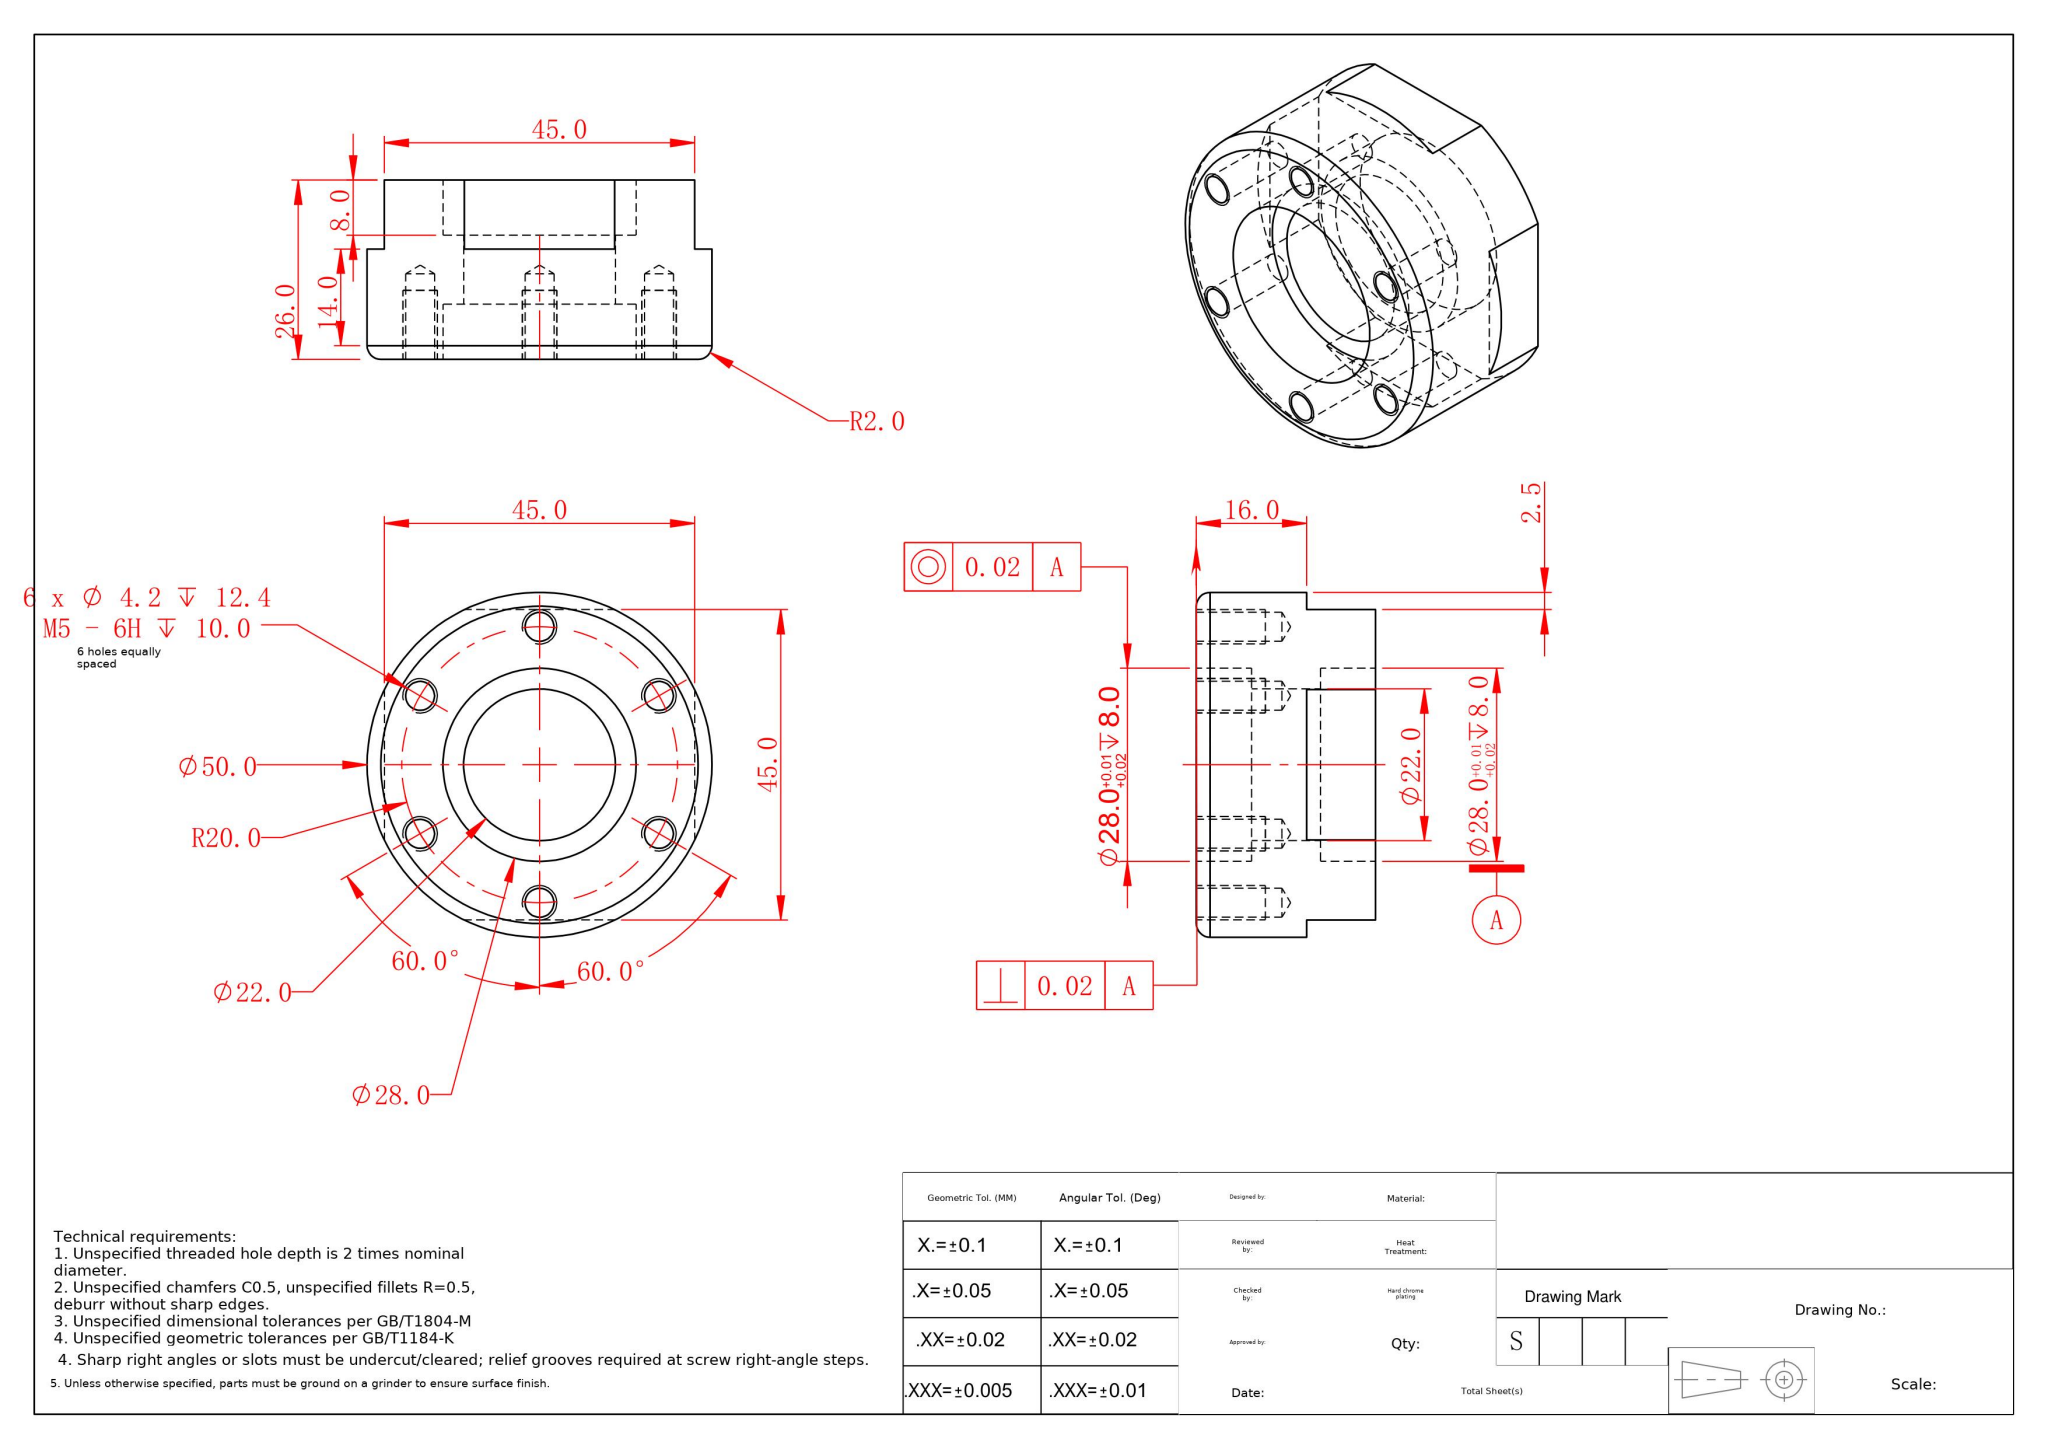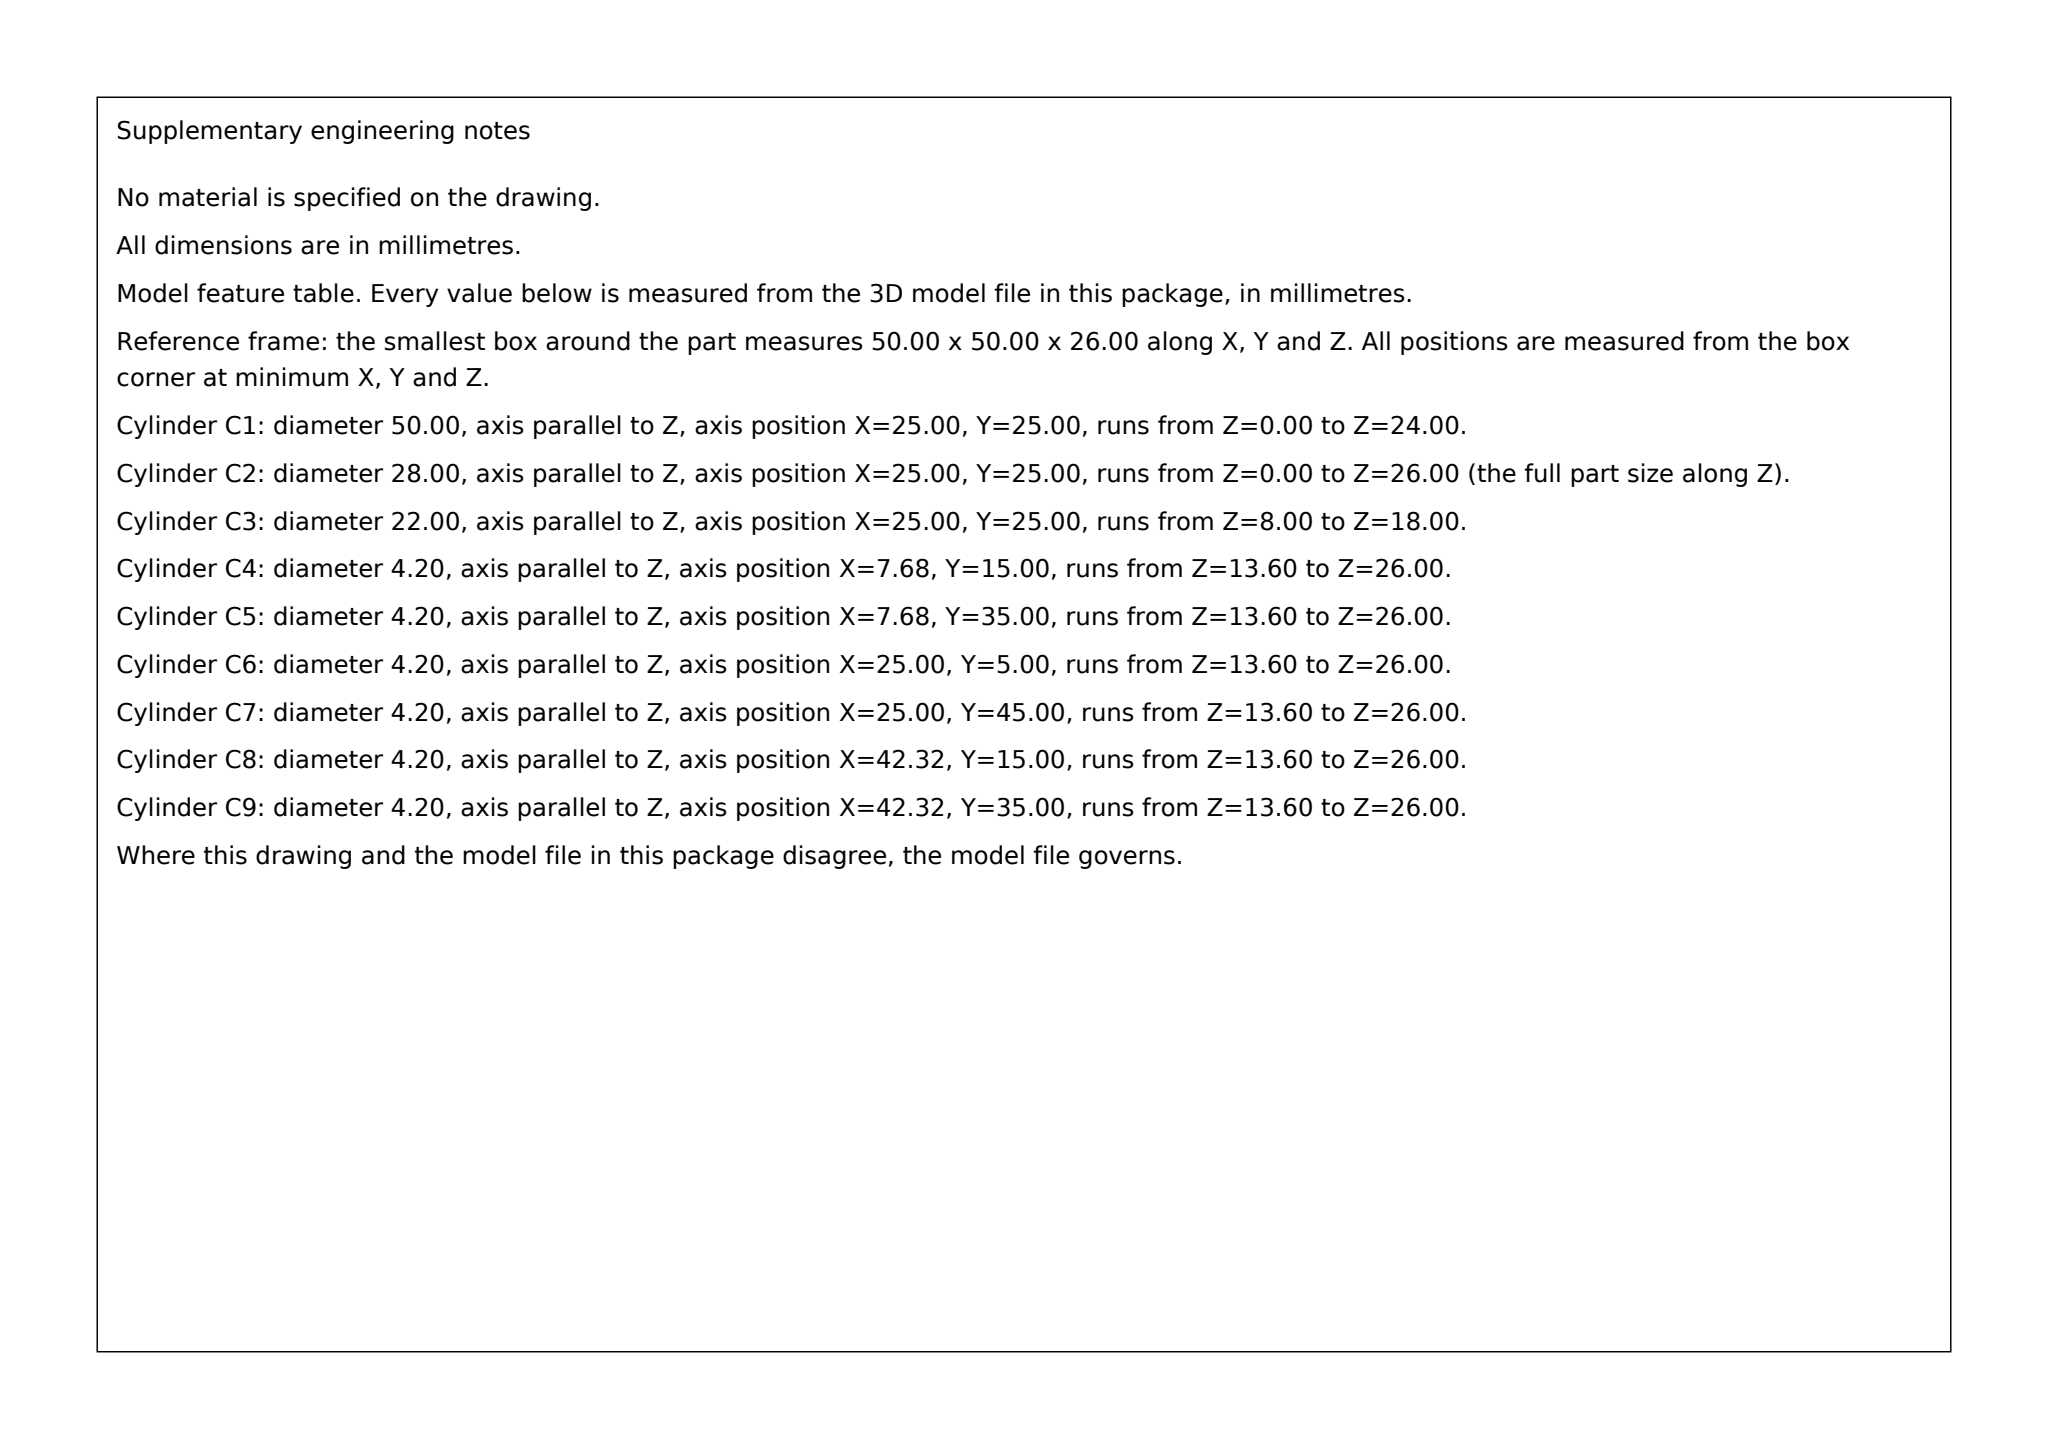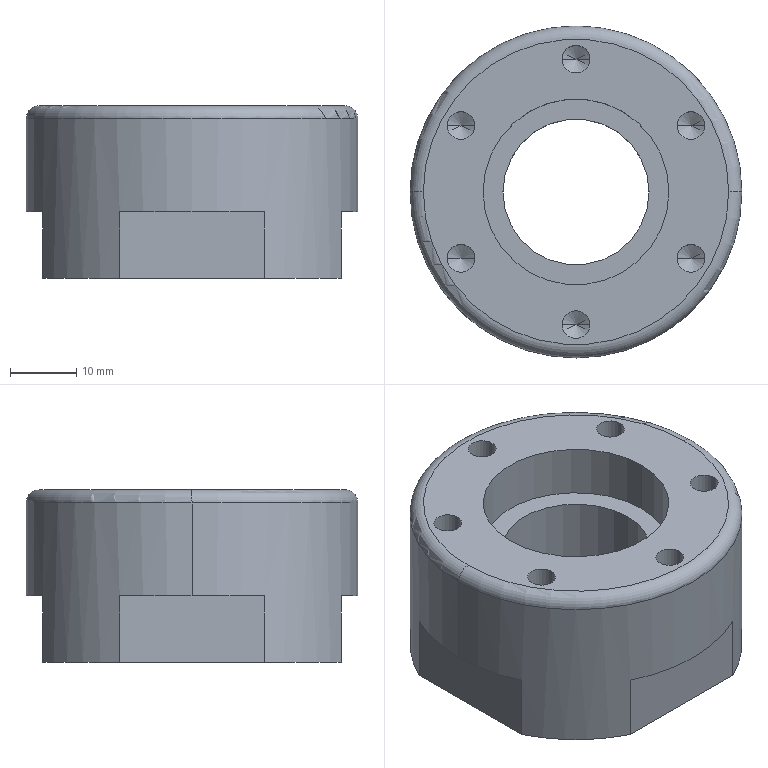Part | SolidWorks | mm | 1 solid | 46 faces | box 50 x 50 x 26 mm | volume 34731 mm3 | cylinder 20 | cone 12 | plane 12 | torus 2 | commonest cylinder face diameters 4.2 x12 28 x4 22 x2 50 x2
build123d program:
from build123d import *

# Parameters (mm, degrees)
SKETCH1_R           = 25
BOSS_EXTRUDE1_DEPTH = 26
SKETCH2_R           = 14
CUT_EXTRUDE1_DEPTH  = 8
CUT_EXTRUDE2_START  = -8
SKETCH3_R           = 14
CUT_EXTRUDE2_DEPTH  = 8
CUT_EXTRUDE3_REACH  = 41.674
SKETCH4_R           = 11
SKETCH6_OUTSIDE_W   = 67.068
SKETCH6_OUTSIDE_H   = 67.068
SKETCH6_OUTSIDE_W_2 = 45
SKETCH6_OUTSIDE_H_2 = 45
CUT_EXTRUDE4_DEPTH  = 10
CIRPATTERN1_COUNT   = 6
FILLET1_R           = 2


with BuildPart() as part:
    # Sketch1 → Boss-Extrude1 (new body)
    with BuildSketch(Plane.XY):
        with Locations(Location((0, 0, 0), (0, 0, 180))):
            Circle(SKETCH1_R)
    extrude(amount=BOSS_EXTRUDE1_DEPTH)

    # Sketch2 → Cut-Extrude1 (cut)
    with BuildSketch(Plane(origin=(0, 0, 0), x_dir=(-1, 0, 0), z_dir=(0, 0, -1))):
        Circle(SKETCH2_R)
    extrude(amount=-CUT_EXTRUDE1_DEPTH, mode=Mode.SUBTRACT)

    # Sketch3 → Cut-Extrude2 (cut)
    with BuildSketch(Plane.XY.offset(26).offset(CUT_EXTRUDE2_START)):
        with Locations(Location((0, 0, 0), (0, 0, 180))):
            Circle(SKETCH3_R)
    extrude(amount=CUT_EXTRUDE2_DEPTH, mode=Mode.SUBTRACT)

    # Sketch4 → Cut-Extrude3 (cut, up to next)
    with BuildSketch(Plane.XY.offset(18), mode=Mode.PRIVATE) as cut_extrude3_sk1:
        Circle(SKETCH4_R)
    cut_extrude3_tool1 = extrude(cut_extrude3_sk1.sketch, amount=-CUT_EXTRUDE3_REACH, mode=Mode.PRIVATE) & part.part
    add(cut_extrude3_tool1.solids().sort_by_distance((0, 0, 18))[0], mode=Mode.SUBTRACT)

    # Sketch6 outside → Cut-Extrude4 (cut)
    with BuildSketch(Plane(origin=(0, 0, 0), x_dir=(-1, 0, 0), z_dir=(0, 0, -1))):
        Rectangle(SKETCH6_OUTSIDE_W, SKETCH6_OUTSIDE_H)
        Rectangle(SKETCH6_OUTSIDE_W_2, SKETCH6_OUTSIDE_H_2, mode=Mode.SUBTRACT)
    extrude(amount=-CUT_EXTRUDE4_DEPTH, mode=Mode.SUBTRACT)

    # Sketch7 → M5 Tapped Hole1 (revolve, cut)
    with BuildSketch(Plane(origin=(0, 20, 26), x_dir=(0, -1, 0), z_dir=(1, 0, 0))):
        Polygon((0, 0), (0, 13.662), (2.1, 12.4), (2.1, 0), align=None)
    m5_tapped_hole1 = revolve(axis=Axis((0, 20, 32.35), (0, 0, -1)), mode=Mode.SUBTRACT)

    # CirPattern1: M5 Tapped Hole1 ×6 about axis
    cirpattern1_axis = Axis((0, 0, 0), (0, 0, 1))
    for i in range(1, CIRPATTERN1_COUNT):
        add(m5_tapped_hole1.rotate(cirpattern1_axis, i * 360 / CIRPATTERN1_COUNT), mode=Mode.SUBTRACT)

    # Fillet1
    fillet1_edges = [part.edges().sort_by_distance(p)[0] for p in [
        (25, 0, 26),
    ]]
    fillet(fillet1_edges, radius=FILLET1_R)


solid = part.part